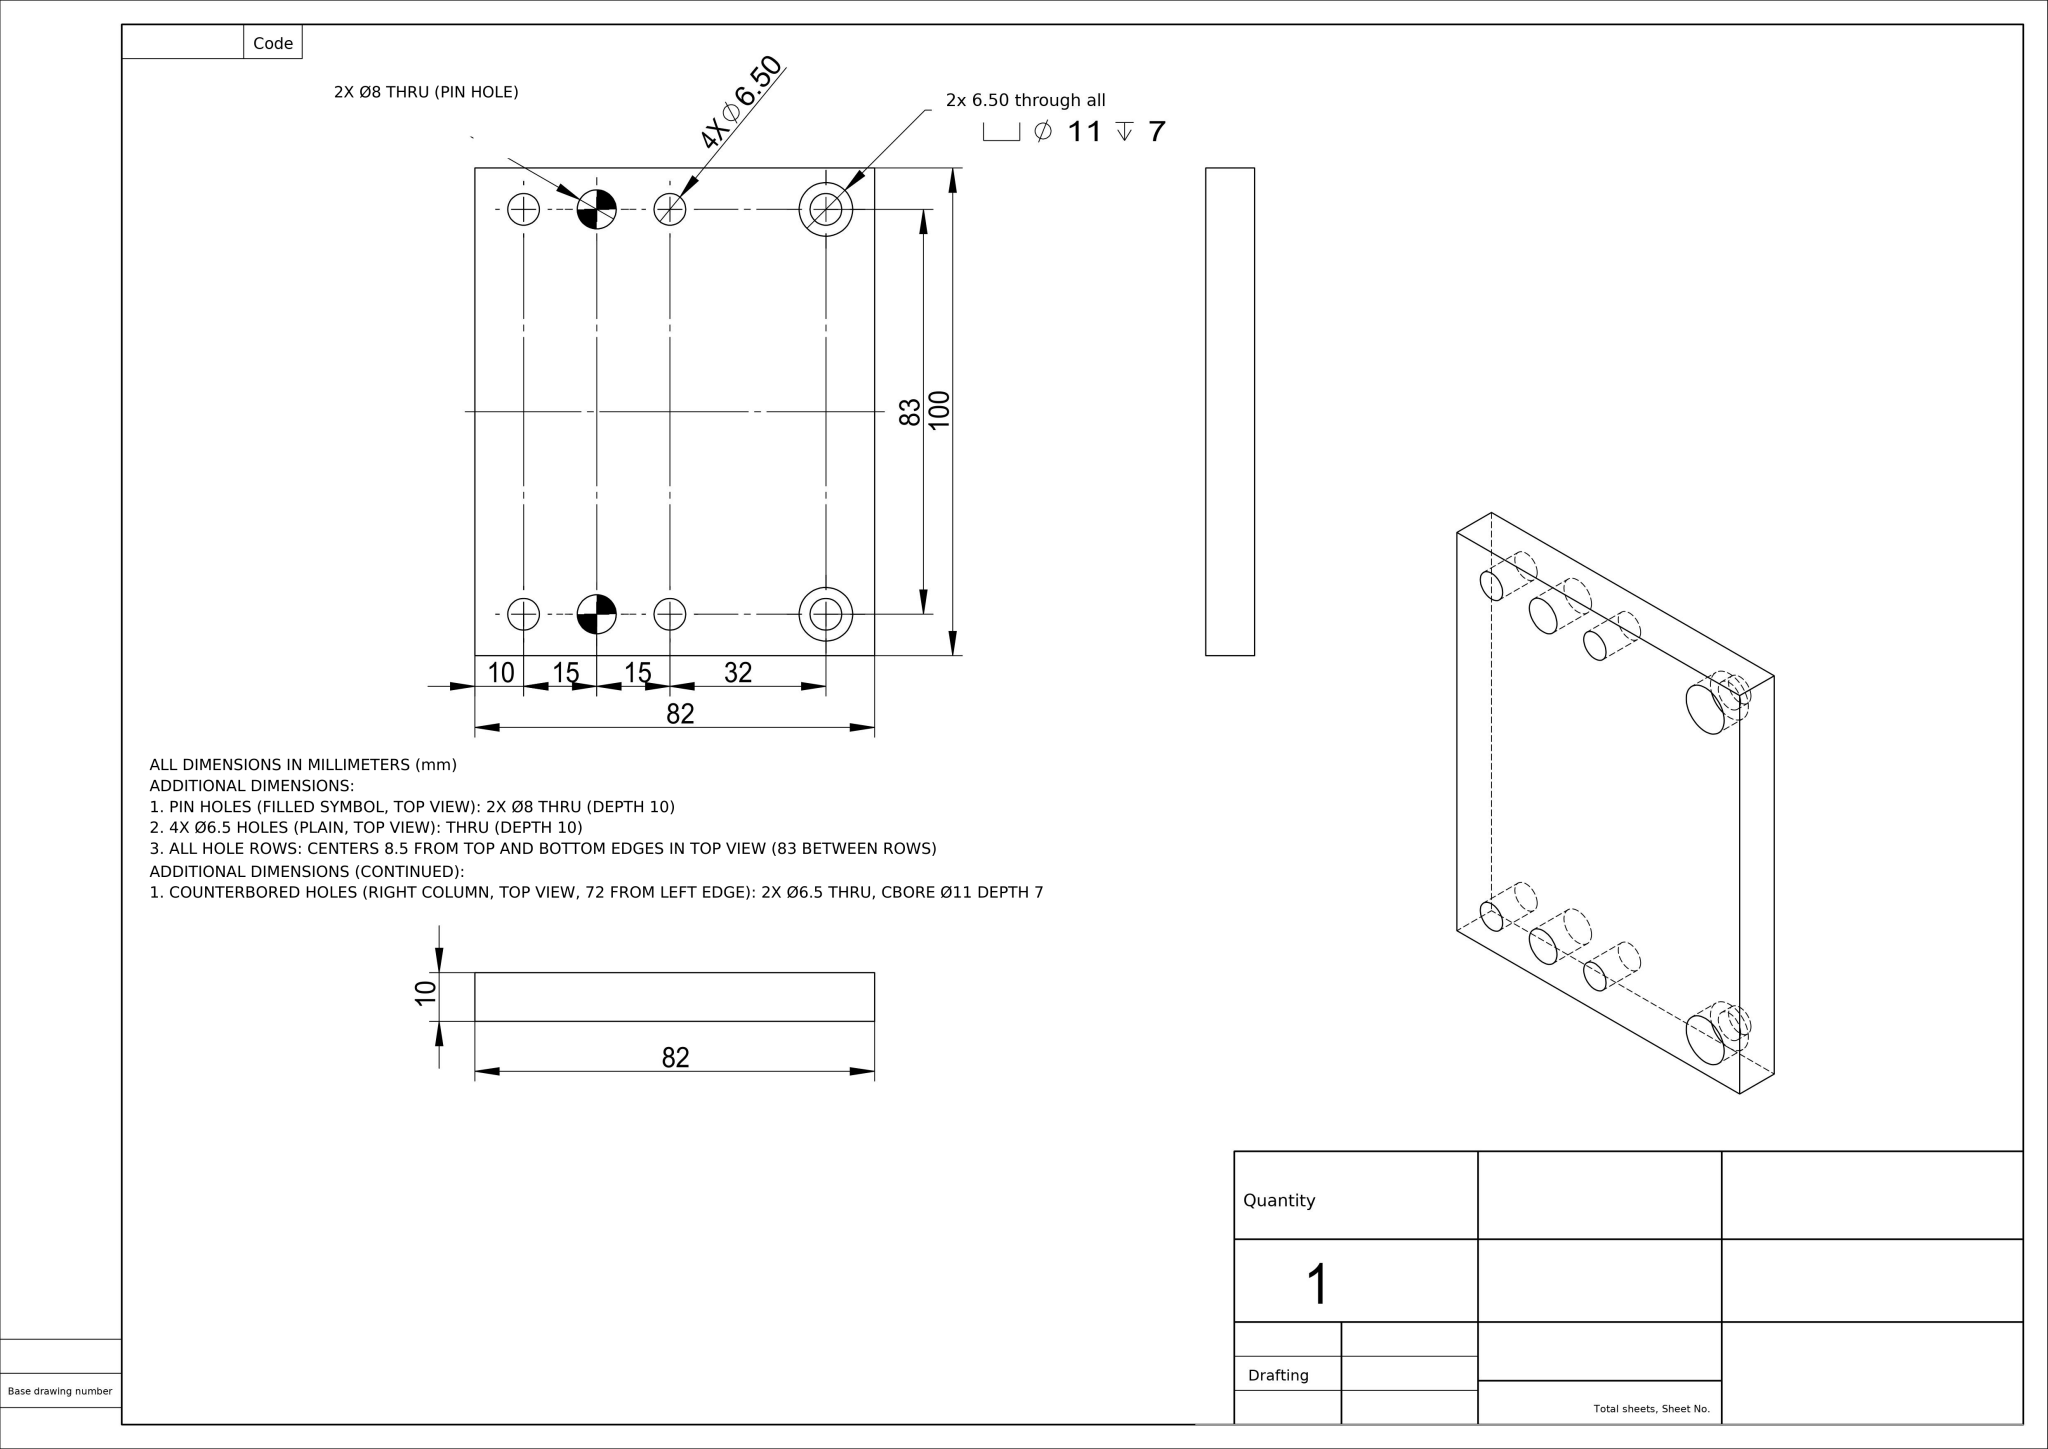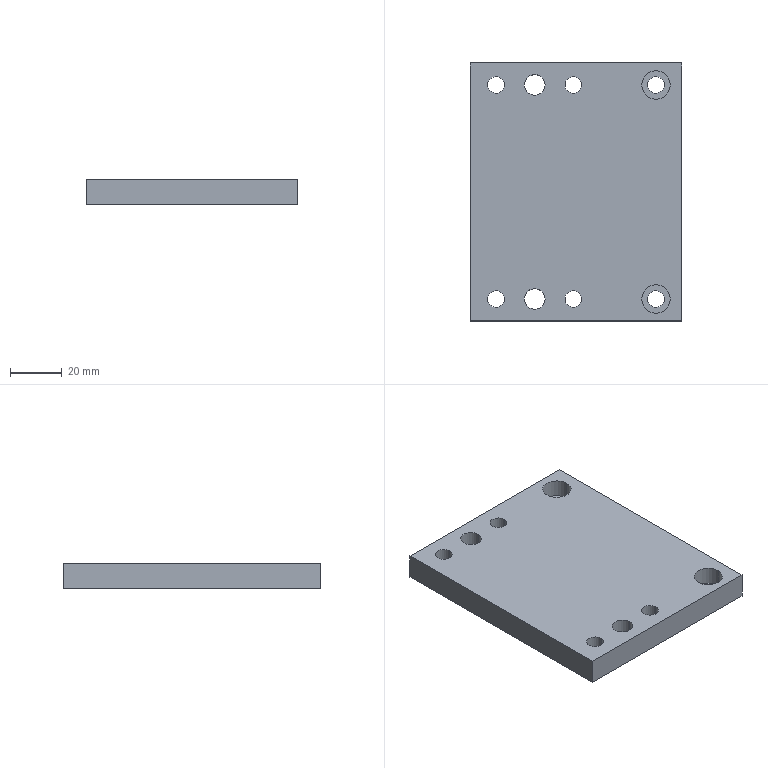Part | NX | mm | 1 solid | 28 faces | box 82 x 100 x 10 mm | volume 78138 mm3 | cylinder 20 | plane 8 | commonest cylinder face diameters 6.5 x12 11 x4 8 x4
STEP:
#1=COLOUR_RGB('',0.502,1.,1.);
#2=FILL_AREA_STYLE_COLOUR('',#1);
#3=FILL_AREA_STYLE('',(#2));
#4=SURFACE_STYLE_FILL_AREA(#3);
#5=SURFACE_SIDE_STYLE('',(#4));
#6=SURFACE_STYLE_USAGE(.BOTH.,#5);
#7=PRESENTATION_STYLE_ASSIGNMENT((#6));
#8=CARTESIAN_POINT('',(25.5,-41.5,-7.));
#9=VERTEX_POINT('',#8);
#10=CARTESIAN_POINT('',(36.5,-41.5,-7.));
#11=VERTEX_POINT('',#10);
#12=CARTESIAN_POINT('',(31.,-41.5,-7.));
#13=DIRECTION('',(0.,0.,1.));
#14=DIRECTION('',(1.,0.,0.));
#15=AXIS2_PLACEMENT_3D('',#12,#13,#14);
#16=CIRCLE('',#15,5.5);
#17=EDGE_CURVE('',#9,#11,#16,.T.);
#18=ORIENTED_EDGE('',*,*,#17,.F.);
#19=CARTESIAN_POINT('',(25.5,-41.5,-0.));
#20=VERTEX_POINT('',#19);
#21=CARTESIAN_POINT('',(25.5,-41.5,0.));
#22=DIRECTION('',(0.,0.,1.));
#23=VECTOR('',#22,1000.);
#24=LINE('',#21,#23);
#25=EDGE_CURVE('',#9,#20,#24,.T.);
#26=ORIENTED_EDGE('',*,*,#25,.T.);
#27=CARTESIAN_POINT('',(36.5,-41.5,-0.));
#28=VERTEX_POINT('',#27);
#29=CARTESIAN_POINT('',(31.,-41.5,-0.));
#30=DIRECTION('',(0.,0.,1.));
#31=DIRECTION('',(1.,0.,0.));
#32=AXIS2_PLACEMENT_3D('',#29,#30,#31);
#33=CIRCLE('',#32,5.5);
#34=EDGE_CURVE('',#20,#28,#33,.T.);
#35=ORIENTED_EDGE('',*,*,#34,.T.);
#36=CARTESIAN_POINT('',(36.5,-41.5,0.));
#37=DIRECTION('',(0.,0.,1.));
#38=VECTOR('',#37,1000.);
#39=LINE('',#36,#38);
#40=EDGE_CURVE('',#11,#28,#39,.T.);
#41=ORIENTED_EDGE('',*,*,#40,.F.);
#42=EDGE_LOOP('',(#18,#26,#35,#41));
#43=FACE_OUTER_BOUND('',#42,.T.);
#44=CARTESIAN_POINT('',(31.,-41.5,0.));
#45=DIRECTION('',(0.,0.,1.));
#46=DIRECTION('',(1.,0.,0.));
#47=AXIS2_PLACEMENT_3D('',#44,#45,#46);
#48=CYLINDRICAL_SURFACE('',#47,5.5);
#49=ADVANCED_FACE('',(#43),#48,.F.);
#50=CARTESIAN_POINT('',(27.75,-41.5,-10.));
#51=VERTEX_POINT('',#50);
#52=CARTESIAN_POINT('',(34.25,-41.5,-10.));
#53=VERTEX_POINT('',#52);
#54=CARTESIAN_POINT('',(31.,-41.5,-10.));
#55=DIRECTION('',(0.,0.,1.));
#56=DIRECTION('',(1.,0.,0.));
#57=AXIS2_PLACEMENT_3D('',#54,#55,#56);
#58=CIRCLE('',#57,3.25);
#59=EDGE_CURVE('',#51,#53,#58,.T.);
#60=ORIENTED_EDGE('',*,*,#59,.F.);
#61=CARTESIAN_POINT('',(27.75,-41.5,-7.));
#62=VERTEX_POINT('',#61);
#63=CARTESIAN_POINT('',(27.75,-41.5,0.));
#64=DIRECTION('',(0.,0.,1.));
#65=VECTOR('',#64,1000.);
#66=LINE('',#63,#65);
#67=EDGE_CURVE('',#51,#62,#66,.T.);
#68=ORIENTED_EDGE('',*,*,#67,.T.);
#69=CARTESIAN_POINT('',(34.25,-41.5,-7.));
#70=VERTEX_POINT('',#69);
#71=CARTESIAN_POINT('',(31.,-41.5,-7.));
#72=DIRECTION('',(0.,0.,1.));
#73=DIRECTION('',(1.,0.,0.));
#74=AXIS2_PLACEMENT_3D('',#71,#72,#73);
#75=CIRCLE('',#74,3.25);
#76=EDGE_CURVE('',#62,#70,#75,.T.);
#77=ORIENTED_EDGE('',*,*,#76,.T.);
#78=CARTESIAN_POINT('',(34.25,-41.5,0.));
#79=DIRECTION('',(0.,0.,1.));
#80=VECTOR('',#79,1000.);
#81=LINE('',#78,#80);
#82=EDGE_CURVE('',#53,#70,#81,.T.);
#83=ORIENTED_EDGE('',*,*,#82,.F.);
#84=EDGE_LOOP('',(#60,#68,#77,#83));
#85=FACE_OUTER_BOUND('',#84,.T.);
#86=CARTESIAN_POINT('',(31.,-41.5,0.));
#87=DIRECTION('',(0.,0.,1.));
#88=DIRECTION('',(1.,0.,0.));
#89=AXIS2_PLACEMENT_3D('',#86,#87,#88);
#90=CYLINDRICAL_SURFACE('',#89,3.25);
#91=ADVANCED_FACE('',(#85),#90,.F.);
#92=CARTESIAN_POINT('',(25.5,41.5,-7.));
#93=VERTEX_POINT('',#92);
#94=CARTESIAN_POINT('',(36.5,41.5,-7.));
#95=VERTEX_POINT('',#94);
#96=CARTESIAN_POINT('',(31.,41.5,-7.));
#97=DIRECTION('',(0.,0.,1.));
#98=DIRECTION('',(1.,0.,0.));
#99=AXIS2_PLACEMENT_3D('',#96,#97,#98);
#100=CIRCLE('',#99,5.5);
#101=EDGE_CURVE('',#93,#95,#100,.T.);
#102=ORIENTED_EDGE('',*,*,#101,.F.);
#103=CARTESIAN_POINT('',(25.5,41.5,-0.));
#104=VERTEX_POINT('',#103);
#105=CARTESIAN_POINT('',(25.5,41.5,0.));
#106=DIRECTION('',(0.,0.,1.));
#107=VECTOR('',#106,1000.);
#108=LINE('',#105,#107);
#109=EDGE_CURVE('',#93,#104,#108,.T.);
#110=ORIENTED_EDGE('',*,*,#109,.T.);
#111=CARTESIAN_POINT('',(36.5,41.5,-0.));
#112=VERTEX_POINT('',#111);
#113=CARTESIAN_POINT('',(31.,41.5,-0.));
#114=DIRECTION('',(0.,0.,1.));
#115=DIRECTION('',(1.,0.,0.));
#116=AXIS2_PLACEMENT_3D('',#113,#114,#115);
#117=CIRCLE('',#116,5.5);
#118=EDGE_CURVE('',#104,#112,#117,.T.);
#119=ORIENTED_EDGE('',*,*,#118,.T.);
#120=CARTESIAN_POINT('',(36.5,41.5,0.));
#121=DIRECTION('',(0.,0.,1.));
#122=VECTOR('',#121,1000.);
#123=LINE('',#120,#122);
#124=EDGE_CURVE('',#95,#112,#123,.T.);
#125=ORIENTED_EDGE('',*,*,#124,.F.);
#126=EDGE_LOOP('',(#102,#110,#119,#125));
#127=FACE_OUTER_BOUND('',#126,.T.);
#128=CARTESIAN_POINT('',(31.,41.5,0.));
#129=DIRECTION('',(0.,0.,1.));
#130=DIRECTION('',(1.,0.,0.));
#131=AXIS2_PLACEMENT_3D('',#128,#129,#130);
#132=CYLINDRICAL_SURFACE('',#131,5.5);
#133=ADVANCED_FACE('',(#127),#132,.F.);
#134=CARTESIAN_POINT('',(27.75,41.5,-10.));
#135=VERTEX_POINT('',#134);
#136=CARTESIAN_POINT('',(34.25,41.5,-10.));
#137=VERTEX_POINT('',#136);
#138=CARTESIAN_POINT('',(31.,41.5,-10.));
#139=DIRECTION('',(0.,0.,1.));
#140=DIRECTION('',(1.,0.,0.));
#141=AXIS2_PLACEMENT_3D('',#138,#139,#140);
#142=CIRCLE('',#141,3.25);
#143=EDGE_CURVE('',#135,#137,#142,.T.);
#144=ORIENTED_EDGE('',*,*,#143,.F.);
#145=CARTESIAN_POINT('',(27.75,41.5,-7.));
#146=VERTEX_POINT('',#145);
#147=CARTESIAN_POINT('',(27.75,41.5,0.));
#148=DIRECTION('',(0.,0.,1.));
#149=VECTOR('',#148,1000.);
#150=LINE('',#147,#149);
#151=EDGE_CURVE('',#135,#146,#150,.T.);
#152=ORIENTED_EDGE('',*,*,#151,.T.);
#153=CARTESIAN_POINT('',(34.25,41.5,-7.));
#154=VERTEX_POINT('',#153);
#155=CARTESIAN_POINT('',(31.,41.5,-7.));
#156=DIRECTION('',(0.,0.,1.));
#157=DIRECTION('',(1.,0.,0.));
#158=AXIS2_PLACEMENT_3D('',#155,#156,#157);
#159=CIRCLE('',#158,3.25);
#160=EDGE_CURVE('',#146,#154,#159,.T.);
#161=ORIENTED_EDGE('',*,*,#160,.T.);
#162=CARTESIAN_POINT('',(34.25,41.5,0.));
#163=DIRECTION('',(0.,0.,1.));
#164=VECTOR('',#163,1000.);
#165=LINE('',#162,#164);
#166=EDGE_CURVE('',#137,#154,#165,.T.);
#167=ORIENTED_EDGE('',*,*,#166,.F.);
#168=EDGE_LOOP('',(#144,#152,#161,#167));
#169=FACE_OUTER_BOUND('',#168,.T.);
#170=CARTESIAN_POINT('',(31.,41.5,0.));
#171=DIRECTION('',(0.,0.,1.));
#172=DIRECTION('',(1.,0.,0.));
#173=AXIS2_PLACEMENT_3D('',#170,#171,#172);
#174=CYLINDRICAL_SURFACE('',#173,3.25);
#175=ADVANCED_FACE('',(#169),#174,.F.);
#176=CARTESIAN_POINT('',(-20.,-41.5,-10.));
#177=VERTEX_POINT('',#176);
#178=CARTESIAN_POINT('',(-12.,-41.5,-10.));
#179=VERTEX_POINT('',#178);
#180=CARTESIAN_POINT('',(-16.,-41.5,-10.));
#181=DIRECTION('',(0.,0.,1.));
#182=DIRECTION('',(1.,0.,0.));
#183=AXIS2_PLACEMENT_3D('',#180,#181,#182);
#184=CIRCLE('',#183,4.);
#185=EDGE_CURVE('',#177,#179,#184,.T.);
#186=ORIENTED_EDGE('',*,*,#185,.F.);
#187=CARTESIAN_POINT('',(-20.,-41.5,0.));
#188=VERTEX_POINT('',#187);
#189=CARTESIAN_POINT('',(-20.,-41.5,0.));
#190=DIRECTION('',(0.,0.,1.));
#191=VECTOR('',#190,1000.);
#192=LINE('',#189,#191);
#193=EDGE_CURVE('',#177,#188,#192,.T.);
#194=ORIENTED_EDGE('',*,*,#193,.T.);
#195=CARTESIAN_POINT('',(-12.,-41.5,0.));
#196=VERTEX_POINT('',#195);
#197=CARTESIAN_POINT('',(-16.,-41.5,0.));
#198=DIRECTION('',(0.,0.,1.));
#199=DIRECTION('',(1.,0.,0.));
#200=AXIS2_PLACEMENT_3D('',#197,#198,#199);
#201=CIRCLE('',#200,4.);
#202=EDGE_CURVE('',#188,#196,#201,.T.);
#203=ORIENTED_EDGE('',*,*,#202,.T.);
#204=CARTESIAN_POINT('',(-12.,-41.5,0.));
#205=DIRECTION('',(0.,0.,1.));
#206=VECTOR('',#205,1000.);
#207=LINE('',#204,#206);
#208=EDGE_CURVE('',#179,#196,#207,.T.);
#209=ORIENTED_EDGE('',*,*,#208,.F.);
#210=EDGE_LOOP('',(#186,#194,#203,#209));
#211=FACE_OUTER_BOUND('',#210,.T.);
#212=CARTESIAN_POINT('',(-16.,-41.5,0.));
#213=DIRECTION('',(0.,0.,1.));
#214=DIRECTION('',(1.,0.,0.));
#215=AXIS2_PLACEMENT_3D('',#212,#213,#214);
#216=CYLINDRICAL_SURFACE('',#215,4.);
#217=ADVANCED_FACE('',(#211),#216,.F.);
#218=CARTESIAN_POINT('',(-20.,41.5,-10.));
#219=VERTEX_POINT('',#218);
#220=CARTESIAN_POINT('',(-12.,41.5,-10.));
#221=VERTEX_POINT('',#220);
#222=CARTESIAN_POINT('',(-16.,41.5,-10.));
#223=DIRECTION('',(0.,0.,1.));
#224=DIRECTION('',(1.,0.,0.));
#225=AXIS2_PLACEMENT_3D('',#222,#223,#224);
#226=CIRCLE('',#225,4.);
#227=EDGE_CURVE('',#219,#221,#226,.T.);
#228=ORIENTED_EDGE('',*,*,#227,.F.);
#229=CARTESIAN_POINT('',(-20.,41.5,0.));
#230=VERTEX_POINT('',#229);
#231=CARTESIAN_POINT('',(-20.,41.5,0.));
#232=DIRECTION('',(0.,0.,1.));
#233=VECTOR('',#232,1000.);
#234=LINE('',#231,#233);
#235=EDGE_CURVE('',#219,#230,#234,.T.);
#236=ORIENTED_EDGE('',*,*,#235,.T.);
#237=CARTESIAN_POINT('',(-12.,41.5,0.));
#238=VERTEX_POINT('',#237);
#239=CARTESIAN_POINT('',(-16.,41.5,0.));
#240=DIRECTION('',(0.,0.,1.));
#241=DIRECTION('',(1.,0.,0.));
#242=AXIS2_PLACEMENT_3D('',#239,#240,#241);
#243=CIRCLE('',#242,4.);
#244=EDGE_CURVE('',#230,#238,#243,.T.);
#245=ORIENTED_EDGE('',*,*,#244,.T.);
#246=CARTESIAN_POINT('',(-12.,41.5,0.));
#247=DIRECTION('',(0.,0.,1.));
#248=VECTOR('',#247,1000.);
#249=LINE('',#246,#248);
#250=EDGE_CURVE('',#221,#238,#249,.T.);
#251=ORIENTED_EDGE('',*,*,#250,.F.);
#252=EDGE_LOOP('',(#228,#236,#245,#251));
#253=FACE_OUTER_BOUND('',#252,.T.);
#254=CARTESIAN_POINT('',(-16.,41.5,0.));
#255=DIRECTION('',(0.,0.,1.));
#256=DIRECTION('',(1.,0.,0.));
#257=AXIS2_PLACEMENT_3D('',#254,#255,#256);
#258=CYLINDRICAL_SURFACE('',#257,4.);
#259=ADVANCED_FACE('',(#253),#258,.F.);
#260=CARTESIAN_POINT('',(-4.25,41.5,-10.));
#261=VERTEX_POINT('',#260);
#262=CARTESIAN_POINT('',(2.25,41.5,-10.));
#263=VERTEX_POINT('',#262);
#264=CARTESIAN_POINT('',(-1.,41.5,-10.));
#265=DIRECTION('',(0.,0.,1.));
#266=DIRECTION('',(1.,0.,0.));
#267=AXIS2_PLACEMENT_3D('',#264,#265,#266);
#268=CIRCLE('',#267,3.25);
#269=EDGE_CURVE('',#261,#263,#268,.T.);
#270=ORIENTED_EDGE('',*,*,#269,.F.);
#271=CARTESIAN_POINT('',(-4.25,41.5,0.));
#272=VERTEX_POINT('',#271);
#273=CARTESIAN_POINT('',(-4.25,41.5,-10.));
#274=DIRECTION('',(0.,0.,1.));
#275=VECTOR('',#274,1000.);
#276=LINE('',#273,#275);
#277=EDGE_CURVE('',#261,#272,#276,.T.);
#278=ORIENTED_EDGE('',*,*,#277,.T.);
#279=CARTESIAN_POINT('',(2.25,41.5,0.));
#280=VERTEX_POINT('',#279);
#281=CARTESIAN_POINT('',(-1.,41.5,0.));
#282=DIRECTION('',(0.,0.,1.));
#283=DIRECTION('',(1.,0.,0.));
#284=AXIS2_PLACEMENT_3D('',#281,#282,#283);
#285=CIRCLE('',#284,3.25);
#286=EDGE_CURVE('',#272,#280,#285,.T.);
#287=ORIENTED_EDGE('',*,*,#286,.T.);
#288=CARTESIAN_POINT('',(2.25,41.5,-10.));
#289=DIRECTION('',(0.,0.,1.));
#290=VECTOR('',#289,1000.);
#291=LINE('',#288,#290);
#292=EDGE_CURVE('',#263,#280,#291,.T.);
#293=ORIENTED_EDGE('',*,*,#292,.F.);
#294=EDGE_LOOP('',(#270,#278,#287,#293));
#295=FACE_OUTER_BOUND('',#294,.T.);
#296=CARTESIAN_POINT('',(-1.,41.5,-10.));
#297=DIRECTION('',(0.,0.,1.));
#298=DIRECTION('',(1.,0.,0.));
#299=AXIS2_PLACEMENT_3D('',#296,#297,#298);
#300=CYLINDRICAL_SURFACE('',#299,3.25);
#301=ADVANCED_FACE('',(#295),#300,.F.);
#302=CARTESIAN_POINT('',(-34.25,41.5,-10.));
#303=VERTEX_POINT('',#302);
#304=CARTESIAN_POINT('',(-27.75,41.5,-10.));
#305=VERTEX_POINT('',#304);
#306=CARTESIAN_POINT('',(-31.,41.5,-10.));
#307=DIRECTION('',(0.,0.,1.));
#308=DIRECTION('',(1.,0.,0.));
#309=AXIS2_PLACEMENT_3D('',#306,#307,#308);
#310=CIRCLE('',#309,3.25);
#311=EDGE_CURVE('',#303,#305,#310,.T.);
#312=ORIENTED_EDGE('',*,*,#311,.F.);
#313=CARTESIAN_POINT('',(-34.25,41.5,0.));
#314=VERTEX_POINT('',#313);
#315=CARTESIAN_POINT('',(-34.25,41.5,-10.));
#316=DIRECTION('',(0.,0.,1.));
#317=VECTOR('',#316,1000.);
#318=LINE('',#315,#317);
#319=EDGE_CURVE('',#303,#314,#318,.T.);
#320=ORIENTED_EDGE('',*,*,#319,.T.);
#321=CARTESIAN_POINT('',(-27.75,41.5,0.));
#322=VERTEX_POINT('',#321);
#323=CARTESIAN_POINT('',(-31.,41.5,0.));
#324=DIRECTION('',(0.,0.,1.));
#325=DIRECTION('',(1.,0.,0.));
#326=AXIS2_PLACEMENT_3D('',#323,#324,#325);
#327=CIRCLE('',#326,3.25);
#328=EDGE_CURVE('',#314,#322,#327,.T.);
#329=ORIENTED_EDGE('',*,*,#328,.T.);
#330=CARTESIAN_POINT('',(-27.75,41.5,-10.));
#331=DIRECTION('',(0.,0.,1.));
#332=VECTOR('',#331,1000.);
#333=LINE('',#330,#332);
#334=EDGE_CURVE('',#305,#322,#333,.T.);
#335=ORIENTED_EDGE('',*,*,#334,.F.);
#336=EDGE_LOOP('',(#312,#320,#329,#335));
#337=FACE_OUTER_BOUND('',#336,.T.);
#338=CARTESIAN_POINT('',(-31.,41.5,-10.));
#339=DIRECTION('',(0.,0.,1.));
#340=DIRECTION('',(1.,0.,0.));
#341=AXIS2_PLACEMENT_3D('',#338,#339,#340);
#342=CYLINDRICAL_SURFACE('',#341,3.25);
#343=ADVANCED_FACE('',(#337),#342,.F.);
#344=CARTESIAN_POINT('',(-4.25,-41.5,-10.));
#345=VERTEX_POINT('',#344);
#346=CARTESIAN_POINT('',(2.25,-41.5,-10.));
#347=VERTEX_POINT('',#346);
#348=CARTESIAN_POINT('',(-1.,-41.5,-10.));
#349=DIRECTION('',(0.,0.,1.));
#350=DIRECTION('',(1.,0.,0.));
#351=AXIS2_PLACEMENT_3D('',#348,#349,#350);
#352=CIRCLE('',#351,3.25);
#353=EDGE_CURVE('',#345,#347,#352,.T.);
#354=ORIENTED_EDGE('',*,*,#353,.F.);
#355=CARTESIAN_POINT('',(-4.25,-41.5,0.));
#356=VERTEX_POINT('',#355);
#357=CARTESIAN_POINT('',(-4.25,-41.5,-10.));
#358=DIRECTION('',(0.,0.,1.));
#359=VECTOR('',#358,1000.);
#360=LINE('',#357,#359);
#361=EDGE_CURVE('',#345,#356,#360,.T.);
#362=ORIENTED_EDGE('',*,*,#361,.T.);
#363=CARTESIAN_POINT('',(2.25,-41.5,0.));
#364=VERTEX_POINT('',#363);
#365=CARTESIAN_POINT('',(-1.,-41.5,0.));
#366=DIRECTION('',(0.,0.,1.));
#367=DIRECTION('',(1.,0.,0.));
#368=AXIS2_PLACEMENT_3D('',#365,#366,#367);
#369=CIRCLE('',#368,3.25);
#370=EDGE_CURVE('',#356,#364,#369,.T.);
#371=ORIENTED_EDGE('',*,*,#370,.T.);
#372=CARTESIAN_POINT('',(2.25,-41.5,-10.));
#373=DIRECTION('',(0.,0.,1.));
#374=VECTOR('',#373,1000.);
#375=LINE('',#372,#374);
#376=EDGE_CURVE('',#347,#364,#375,.T.);
#377=ORIENTED_EDGE('',*,*,#376,.F.);
#378=EDGE_LOOP('',(#354,#362,#371,#377));
#379=FACE_OUTER_BOUND('',#378,.T.);
#380=CARTESIAN_POINT('',(-1.,-41.5,-10.));
#381=DIRECTION('',(0.,0.,1.));
#382=DIRECTION('',(1.,0.,0.));
#383=AXIS2_PLACEMENT_3D('',#380,#381,#382);
#384=CYLINDRICAL_SURFACE('',#383,3.25);
#385=ADVANCED_FACE('',(#379),#384,.F.);
#386=CARTESIAN_POINT('',(-34.25,-41.5,-10.));
#387=VERTEX_POINT('',#386);
#388=CARTESIAN_POINT('',(-27.75,-41.5,-10.));
#389=VERTEX_POINT('',#388);
#390=CARTESIAN_POINT('',(-31.,-41.5,-10.));
#391=DIRECTION('',(0.,0.,1.));
#392=DIRECTION('',(1.,0.,0.));
#393=AXIS2_PLACEMENT_3D('',#390,#391,#392);
#394=CIRCLE('',#393,3.25);
#395=EDGE_CURVE('',#387,#389,#394,.T.);
#396=ORIENTED_EDGE('',*,*,#395,.F.);
#397=CARTESIAN_POINT('',(-34.25,-41.5,0.));
#398=VERTEX_POINT('',#397);
#399=CARTESIAN_POINT('',(-34.25,-41.5,-10.));
#400=DIRECTION('',(0.,0.,1.));
#401=VECTOR('',#400,1000.);
#402=LINE('',#399,#401);
#403=EDGE_CURVE('',#387,#398,#402,.T.);
#404=ORIENTED_EDGE('',*,*,#403,.T.);
#405=CARTESIAN_POINT('',(-27.75,-41.5,0.));
#406=VERTEX_POINT('',#405);
#407=CARTESIAN_POINT('',(-31.,-41.5,0.));
#408=DIRECTION('',(0.,0.,1.));
#409=DIRECTION('',(1.,0.,0.));
#410=AXIS2_PLACEMENT_3D('',#407,#408,#409);
#411=CIRCLE('',#410,3.25);
#412=EDGE_CURVE('',#398,#406,#411,.T.);
#413=ORIENTED_EDGE('',*,*,#412,.T.);
#414=CARTESIAN_POINT('',(-27.75,-41.5,-10.));
#415=DIRECTION('',(0.,0.,1.));
#416=VECTOR('',#415,1000.);
#417=LINE('',#414,#416);
#418=EDGE_CURVE('',#389,#406,#417,.T.);
#419=ORIENTED_EDGE('',*,*,#418,.F.);
#420=EDGE_LOOP('',(#396,#404,#413,#419));
#421=FACE_OUTER_BOUND('',#420,.T.);
#422=CARTESIAN_POINT('',(-31.,-41.5,-10.));
#423=DIRECTION('',(0.,0.,1.));
#424=DIRECTION('',(1.,0.,0.));
#425=AXIS2_PLACEMENT_3D('',#422,#423,#424);
#426=CYLINDRICAL_SURFACE('',#425,3.25);
#427=ADVANCED_FACE('',(#421),#426,.F.);
#428=CARTESIAN_POINT('',(-41.,50.,0.));
#429=VERTEX_POINT('',#428);
#430=CARTESIAN_POINT('',(-41.,-50.,0.));
#431=VERTEX_POINT('',#430);
#432=CARTESIAN_POINT('',(-41.,50.,0.));
#433=DIRECTION('',(0.,-1.,0.));
#434=VECTOR('',#433,1000.);
#435=LINE('',#432,#434);
#436=EDGE_CURVE('',#429,#431,#435,.T.);
#437=ORIENTED_EDGE('',*,*,#436,.F.);
#438=CARTESIAN_POINT('',(-41.,50.,-10.));
#439=VERTEX_POINT('',#438);
#440=CARTESIAN_POINT('',(-41.,50.,-10.));
#441=DIRECTION('',(0.,0.,1.));
#442=VECTOR('',#441,1000.);
#443=LINE('',#440,#442);
#444=EDGE_CURVE('',#439,#429,#443,.T.);
#445=ORIENTED_EDGE('',*,*,#444,.F.);
#446=CARTESIAN_POINT('',(-41.,-50.,-10.));
#447=VERTEX_POINT('',#446);
#448=CARTESIAN_POINT('',(-41.,50.,-10.));
#449=DIRECTION('',(0.,-1.,0.));
#450=VECTOR('',#449,1000.);
#451=LINE('',#448,#450);
#452=EDGE_CURVE('',#439,#447,#451,.T.);
#453=ORIENTED_EDGE('',*,*,#452,.T.);
#454=CARTESIAN_POINT('',(-41.,-50.,-10.));
#455=DIRECTION('',(0.,0.,1.));
#456=VECTOR('',#455,1000.);
#457=LINE('',#454,#456);
#458=EDGE_CURVE('',#447,#431,#457,.T.);
#459=ORIENTED_EDGE('',*,*,#458,.T.);
#460=EDGE_LOOP('',(#437,#445,#453,#459));
#461=FACE_OUTER_BOUND('',#460,.T.);
#462=CARTESIAN_POINT('',(-41.,50.,-10.));
#463=DIRECTION('',(-1.,0.,0.));
#464=DIRECTION('',(0.,0.,1.));
#465=AXIS2_PLACEMENT_3D('',#462,#463,#464);
#466=PLANE('',#465);
#467=ADVANCED_FACE('',(#461),#466,.T.);
#468=CARTESIAN_POINT('',(41.,50.,0.));
#469=VERTEX_POINT('',#468);
#470=CARTESIAN_POINT('',(-41.,50.,0.));
#471=DIRECTION('',(-1.,0.,0.));
#472=VECTOR('',#471,1000.);
#473=LINE('',#470,#472);
#474=EDGE_CURVE('',#469,#429,#473,.T.);
#475=ORIENTED_EDGE('',*,*,#474,.F.);
#476=CARTESIAN_POINT('',(41.,50.,-10.));
#477=VERTEX_POINT('',#476);
#478=CARTESIAN_POINT('',(41.,50.,-10.));
#479=DIRECTION('',(0.,0.,1.));
#480=VECTOR('',#479,1000.);
#481=LINE('',#478,#480);
#482=EDGE_CURVE('',#477,#469,#481,.T.);
#483=ORIENTED_EDGE('',*,*,#482,.F.);
#484=CARTESIAN_POINT('',(-41.,50.,-10.));
#485=DIRECTION('',(-1.,0.,0.));
#486=VECTOR('',#485,1000.);
#487=LINE('',#484,#486);
#488=EDGE_CURVE('',#477,#439,#487,.T.);
#489=ORIENTED_EDGE('',*,*,#488,.T.);
#490=ORIENTED_EDGE('',*,*,#444,.T.);
#491=EDGE_LOOP('',(#475,#483,#489,#490));
#492=FACE_OUTER_BOUND('',#491,.T.);
#493=CARTESIAN_POINT('',(-41.,50.,-10.));
#494=DIRECTION('',(0.,1.,0.));
#495=DIRECTION('',(0.,0.,1.));
#496=AXIS2_PLACEMENT_3D('',#493,#494,#495);
#497=PLANE('',#496);
#498=ADVANCED_FACE('',(#492),#497,.T.);
#499=CARTESIAN_POINT('',(41.,-50.,0.));
#500=VERTEX_POINT('',#499);
#501=CARTESIAN_POINT('',(41.,50.,0.));
#502=DIRECTION('',(0.,1.,0.));
#503=VECTOR('',#502,1000.);
#504=LINE('',#501,#503);
#505=EDGE_CURVE('',#500,#469,#504,.T.);
#506=ORIENTED_EDGE('',*,*,#505,.F.);
#507=CARTESIAN_POINT('',(41.,-50.,-10.));
#508=VERTEX_POINT('',#507);
#509=CARTESIAN_POINT('',(41.,-50.,-10.));
#510=DIRECTION('',(0.,0.,1.));
#511=VECTOR('',#510,1000.);
#512=LINE('',#509,#511);
#513=EDGE_CURVE('',#508,#500,#512,.T.);
#514=ORIENTED_EDGE('',*,*,#513,.F.);
#515=CARTESIAN_POINT('',(41.,50.,-10.));
#516=DIRECTION('',(0.,1.,0.));
#517=VECTOR('',#516,1000.);
#518=LINE('',#515,#517);
#519=EDGE_CURVE('',#508,#477,#518,.T.);
#520=ORIENTED_EDGE('',*,*,#519,.T.);
#521=ORIENTED_EDGE('',*,*,#482,.T.);
#522=EDGE_LOOP('',(#506,#514,#520,#521));
#523=FACE_OUTER_BOUND('',#522,.T.);
#524=CARTESIAN_POINT('',(41.,50.,-10.));
#525=DIRECTION('',(1.,0.,0.));
#526=DIRECTION('',(0.,0.,-1.));
#527=AXIS2_PLACEMENT_3D('',#524,#525,#526);
#528=PLANE('',#527);
#529=ADVANCED_FACE('',(#523),#528,.T.);
#530=CARTESIAN_POINT('',(-41.,-50.,0.));
#531=DIRECTION('',(1.,0.,0.));
#532=VECTOR('',#531,1000.);
#533=LINE('',#530,#532);
#534=EDGE_CURVE('',#431,#500,#533,.T.);
#535=ORIENTED_EDGE('',*,*,#534,.F.);
#536=ORIENTED_EDGE('',*,*,#458,.F.);
#537=CARTESIAN_POINT('',(-41.,-50.,-10.));
#538=DIRECTION('',(1.,0.,0.));
#539=VECTOR('',#538,1000.);
#540=LINE('',#537,#539);
#541=EDGE_CURVE('',#447,#508,#540,.T.);
#542=ORIENTED_EDGE('',*,*,#541,.T.);
#543=ORIENTED_EDGE('',*,*,#513,.T.);
#544=EDGE_LOOP('',(#535,#536,#542,#543));
#545=FACE_OUTER_BOUND('',#544,.T.);
#546=CARTESIAN_POINT('',(-41.,-50.,-10.));
#547=DIRECTION('',(0.,-1.,0.));
#548=DIRECTION('',(0.,0.,-1.));
#549=AXIS2_PLACEMENT_3D('',#546,#547,#548);
#550=PLANE('',#549);
#551=ADVANCED_FACE('',(#545),#550,.T.);
#552=CARTESIAN_POINT('',(31.,-41.5,-10.));
#553=DIRECTION('',(0.,0.,1.));
#554=DIRECTION('',(1.,0.,0.));
#555=AXIS2_PLACEMENT_3D('',#552,#553,#554);
#556=CIRCLE('',#555,3.25);
#557=EDGE_CURVE('',#53,#51,#556,.T.);
#558=ORIENTED_EDGE('',*,*,#557,.T.);
#559=ORIENTED_EDGE('',*,*,#59,.T.);
#560=EDGE_LOOP('',(#558,#559));
#561=FACE_BOUND('',#560,.T.);
#562=CARTESIAN_POINT('',(31.,41.5,-10.));
#563=DIRECTION('',(0.,0.,1.));
#564=DIRECTION('',(1.,0.,0.));
#565=AXIS2_PLACEMENT_3D('',#562,#563,#564);
#566=CIRCLE('',#565,3.25);
#567=EDGE_CURVE('',#137,#135,#566,.T.);
#568=ORIENTED_EDGE('',*,*,#567,.T.);
#569=ORIENTED_EDGE('',*,*,#143,.T.);
#570=EDGE_LOOP('',(#568,#569));
#571=FACE_BOUND('',#570,.T.);
#572=CARTESIAN_POINT('',(-16.,-41.5,-10.));
#573=DIRECTION('',(0.,0.,1.));
#574=DIRECTION('',(1.,0.,0.));
#575=AXIS2_PLACEMENT_3D('',#572,#573,#574);
#576=CIRCLE('',#575,4.);
#577=EDGE_CURVE('',#179,#177,#576,.T.);
#578=ORIENTED_EDGE('',*,*,#577,.T.);
#579=ORIENTED_EDGE('',*,*,#185,.T.);
#580=EDGE_LOOP('',(#578,#579));
#581=FACE_BOUND('',#580,.T.);
#582=CARTESIAN_POINT('',(-16.,41.5,-10.));
#583=DIRECTION('',(0.,0.,1.));
#584=DIRECTION('',(1.,0.,0.));
#585=AXIS2_PLACEMENT_3D('',#582,#583,#584);
#586=CIRCLE('',#585,4.);
#587=EDGE_CURVE('',#221,#219,#586,.T.);
#588=ORIENTED_EDGE('',*,*,#587,.T.);
#589=ORIENTED_EDGE('',*,*,#227,.T.);
#590=EDGE_LOOP('',(#588,#589));
#591=FACE_BOUND('',#590,.T.);
#592=CARTESIAN_POINT('',(-1.,41.5,-10.));
#593=DIRECTION('',(0.,0.,1.));
#594=DIRECTION('',(1.,0.,0.));
#595=AXIS2_PLACEMENT_3D('',#592,#593,#594);
#596=CIRCLE('',#595,3.25);
#597=EDGE_CURVE('',#263,#261,#596,.T.);
#598=ORIENTED_EDGE('',*,*,#597,.T.);
#599=ORIENTED_EDGE('',*,*,#269,.T.);
#600=EDGE_LOOP('',(#598,#599));
#601=FACE_BOUND('',#600,.T.);
#602=CARTESIAN_POINT('',(-31.,41.5,-10.));
#603=DIRECTION('',(0.,0.,1.));
#604=DIRECTION('',(1.,0.,0.));
#605=AXIS2_PLACEMENT_3D('',#602,#603,#604);
#606=CIRCLE('',#605,3.25);
#607=EDGE_CURVE('',#305,#303,#606,.T.);
#608=ORIENTED_EDGE('',*,*,#607,.T.);
#609=ORIENTED_EDGE('',*,*,#311,.T.);
#610=EDGE_LOOP('',(#608,#609));
#611=FACE_BOUND('',#610,.T.);
#612=CARTESIAN_POINT('',(-1.,-41.5,-10.));
#613=DIRECTION('',(0.,0.,1.));
#614=DIRECTION('',(1.,0.,0.));
#615=AXIS2_PLACEMENT_3D('',#612,#613,#614);
#616=CIRCLE('',#615,3.25);
#617=EDGE_CURVE('',#347,#345,#616,.T.);
#618=ORIENTED_EDGE('',*,*,#617,.T.);
#619=ORIENTED_EDGE('',*,*,#353,.T.);
#620=EDGE_LOOP('',(#618,#619));
#621=FACE_BOUND('',#620,.T.);
#622=CARTESIAN_POINT('',(-31.,-41.5,-10.));
#623=DIRECTION('',(0.,0.,1.));
#624=DIRECTION('',(1.,0.,0.));
#625=AXIS2_PLACEMENT_3D('',#622,#623,#624);
#626=CIRCLE('',#625,3.25);
#627=EDGE_CURVE('',#389,#387,#626,.T.);
#628=ORIENTED_EDGE('',*,*,#627,.T.);
#629=ORIENTED_EDGE('',*,*,#395,.T.);
#630=EDGE_LOOP('',(#628,#629));
#631=FACE_BOUND('',#630,.T.);
#632=ORIENTED_EDGE('',*,*,#452,.F.);
#633=ORIENTED_EDGE('',*,*,#488,.F.);
#634=ORIENTED_EDGE('',*,*,#519,.F.);
#635=ORIENTED_EDGE('',*,*,#541,.F.);
#636=EDGE_LOOP('',(#632,#633,#634,#635));
#637=FACE_OUTER_BOUND('',#636,.T.);
#638=CARTESIAN_POINT('',(0.,0.,-10.));
#639=DIRECTION('',(0.,0.,1.));
#640=DIRECTION('',(1.,0.,0.));
#641=AXIS2_PLACEMENT_3D('',#638,#639,#640);
#642=PLANE('',#641);
#643=ADVANCED_FACE('',(#561,#571,#581,#591,#601,#611,#621,#631,#637),#642,.F.);
#644=CARTESIAN_POINT('',(31.,-41.5,-0.));
#645=DIRECTION('',(0.,0.,1.));
#646=DIRECTION('',(1.,0.,0.));
#647=AXIS2_PLACEMENT_3D('',#644,#645,#646);
#648=CIRCLE('',#647,5.5);
#649=EDGE_CURVE('',#28,#20,#648,.T.);
#650=ORIENTED_EDGE('',*,*,#649,.F.);
#651=ORIENTED_EDGE('',*,*,#34,.F.);
#652=EDGE_LOOP('',(#650,#651));
#653=FACE_BOUND('',#652,.T.);
#654=CARTESIAN_POINT('',(31.,41.5,-0.));
#655=DIRECTION('',(0.,0.,1.));
#656=DIRECTION('',(1.,0.,0.));
#657=AXIS2_PLACEMENT_3D('',#654,#655,#656);
#658=CIRCLE('',#657,5.5);
#659=EDGE_CURVE('',#112,#104,#658,.T.);
#660=ORIENTED_EDGE('',*,*,#659,.F.);
#661=ORIENTED_EDGE('',*,*,#118,.F.);
#662=EDGE_LOOP('',(#660,#661));
#663=FACE_BOUND('',#662,.T.);
#664=CARTESIAN_POINT('',(-16.,-41.5,0.));
#665=DIRECTION('',(0.,0.,1.));
#666=DIRECTION('',(1.,0.,0.));
#667=AXIS2_PLACEMENT_3D('',#664,#665,#666);
#668=CIRCLE('',#667,4.);
#669=EDGE_CURVE('',#196,#188,#668,.T.);
#670=ORIENTED_EDGE('',*,*,#669,.F.);
#671=ORIENTED_EDGE('',*,*,#202,.F.);
#672=EDGE_LOOP('',(#670,#671));
#673=FACE_BOUND('',#672,.T.);
#674=CARTESIAN_POINT('',(-16.,41.5,0.));
#675=DIRECTION('',(0.,0.,1.));
#676=DIRECTION('',(1.,0.,0.));
#677=AXIS2_PLACEMENT_3D('',#674,#675,#676);
#678=CIRCLE('',#677,4.);
#679=EDGE_CURVE('',#238,#230,#678,.T.);
#680=ORIENTED_EDGE('',*,*,#679,.F.);
#681=ORIENTED_EDGE('',*,*,#244,.F.);
#682=EDGE_LOOP('',(#680,#681));
#683=FACE_BOUND('',#682,.T.);
#684=CARTESIAN_POINT('',(-1.,41.5,0.));
#685=DIRECTION('',(0.,0.,1.));
#686=DIRECTION('',(1.,0.,0.));
#687=AXIS2_PLACEMENT_3D('',#684,#685,#686);
#688=CIRCLE('',#687,3.25);
#689=EDGE_CURVE('',#280,#272,#688,.T.);
#690=ORIENTED_EDGE('',*,*,#689,.F.);
#691=ORIENTED_EDGE('',*,*,#286,.F.);
#692=EDGE_LOOP('',(#690,#691));
#693=FACE_BOUND('',#692,.T.);
#694=CARTESIAN_POINT('',(-31.,41.5,0.));
#695=DIRECTION('',(0.,0.,1.));
#696=DIRECTION('',(1.,0.,0.));
#697=AXIS2_PLACEMENT_3D('',#694,#695,#696);
#698=CIRCLE('',#697,3.25);
#699=EDGE_CURVE('',#322,#314,#698,.T.);
#700=ORIENTED_EDGE('',*,*,#699,.F.);
#701=ORIENTED_EDGE('',*,*,#328,.F.);
#702=EDGE_LOOP('',(#700,#701));
#703=FACE_BOUND('',#702,.T.);
#704=CARTESIAN_POINT('',(-1.,-41.5,0.));
#705=DIRECTION('',(0.,0.,1.));
#706=DIRECTION('',(1.,0.,0.));
#707=AXIS2_PLACEMENT_3D('',#704,#705,#706);
#708=CIRCLE('',#707,3.25);
#709=EDGE_CURVE('',#364,#356,#708,.T.);
#710=ORIENTED_EDGE('',*,*,#709,.F.);
#711=ORIENTED_EDGE('',*,*,#370,.F.);
#712=EDGE_LOOP('',(#710,#711));
#713=FACE_BOUND('',#712,.T.);
#714=CARTESIAN_POINT('',(-31.,-41.5,0.));
#715=DIRECTION('',(0.,0.,1.));
#716=DIRECTION('',(1.,0.,0.));
#717=AXIS2_PLACEMENT_3D('',#714,#715,#716);
#718=CIRCLE('',#717,3.25);
#719=EDGE_CURVE('',#406,#398,#718,.T.);
#720=ORIENTED_EDGE('',*,*,#719,.F.);
#721=ORIENTED_EDGE('',*,*,#412,.F.);
#722=EDGE_LOOP('',(#720,#721));
#723=FACE_BOUND('',#722,.T.);
#724=ORIENTED_EDGE('',*,*,#436,.T.);
#725=ORIENTED_EDGE('',*,*,#534,.T.);
#726=ORIENTED_EDGE('',*,*,#505,.T.);
#727=ORIENTED_EDGE('',*,*,#474,.T.);
#728=EDGE_LOOP('',(#724,#725,#726,#727));
#729=FACE_OUTER_BOUND('',#728,.T.);
#730=CARTESIAN_POINT('',(0.,0.,0.));
#731=DIRECTION('',(0.,0.,1.));
#732=DIRECTION('',(1.,0.,0.));
#733=AXIS2_PLACEMENT_3D('',#730,#731,#732);
#734=PLANE('',#733);
#735=ADVANCED_FACE('',(#653,#663,#673,#683,#693,#703,#713,#723,#729),#734,.T.);
#736=ORIENTED_EDGE('',*,*,#403,.F.);
#737=ORIENTED_EDGE('',*,*,#627,.F.);
#738=ORIENTED_EDGE('',*,*,#418,.T.);
#739=ORIENTED_EDGE('',*,*,#719,.T.);
#740=EDGE_LOOP('',(#736,#737,#738,#739));
#741=FACE_OUTER_BOUND('',#740,.T.);
#742=CARTESIAN_POINT('',(-31.,-41.5,-10.));
#743=DIRECTION('',(0.,0.,1.));
#744=DIRECTION('',(1.,0.,0.));
#745=AXIS2_PLACEMENT_3D('',#742,#743,#744);
#746=CYLINDRICAL_SURFACE('',#745,3.25);
#747=ADVANCED_FACE('',(#741),#746,.F.);
#748=ORIENTED_EDGE('',*,*,#361,.F.);
#749=ORIENTED_EDGE('',*,*,#617,.F.);
#750=ORIENTED_EDGE('',*,*,#376,.T.);
#751=ORIENTED_EDGE('',*,*,#709,.T.);
#752=EDGE_LOOP('',(#748,#749,#750,#751));
#753=FACE_OUTER_BOUND('',#752,.T.);
#754=CARTESIAN_POINT('',(-1.,-41.5,-10.));
#755=DIRECTION('',(0.,0.,1.));
#756=DIRECTION('',(1.,0.,0.));
#757=AXIS2_PLACEMENT_3D('',#754,#755,#756);
#758=CYLINDRICAL_SURFACE('',#757,3.25);
#759=ADVANCED_FACE('',(#753),#758,.F.);
#760=ORIENTED_EDGE('',*,*,#319,.F.);
#761=ORIENTED_EDGE('',*,*,#607,.F.);
#762=ORIENTED_EDGE('',*,*,#334,.T.);
#763=ORIENTED_EDGE('',*,*,#699,.T.);
#764=EDGE_LOOP('',(#760,#761,#762,#763));
#765=FACE_OUTER_BOUND('',#764,.T.);
#766=CARTESIAN_POINT('',(-31.,41.5,-10.));
#767=DIRECTION('',(0.,0.,1.));
#768=DIRECTION('',(1.,0.,0.));
#769=AXIS2_PLACEMENT_3D('',#766,#767,#768);
#770=CYLINDRICAL_SURFACE('',#769,3.25);
#771=ADVANCED_FACE('',(#765),#770,.F.);
#772=ORIENTED_EDGE('',*,*,#277,.F.);
#773=ORIENTED_EDGE('',*,*,#597,.F.);
#774=ORIENTED_EDGE('',*,*,#292,.T.);
#775=ORIENTED_EDGE('',*,*,#689,.T.);
#776=EDGE_LOOP('',(#772,#773,#774,#775));
#777=FACE_OUTER_BOUND('',#776,.T.);
#778=CARTESIAN_POINT('',(-1.,41.5,-10.));
#779=DIRECTION('',(0.,0.,1.));
#780=DIRECTION('',(1.,0.,0.));
#781=AXIS2_PLACEMENT_3D('',#778,#779,#780);
#782=CYLINDRICAL_SURFACE('',#781,3.25);
#783=ADVANCED_FACE('',(#777),#782,.F.);
#784=ORIENTED_EDGE('',*,*,#235,.F.);
#785=ORIENTED_EDGE('',*,*,#587,.F.);
#786=ORIENTED_EDGE('',*,*,#250,.T.);
#787=ORIENTED_EDGE('',*,*,#679,.T.);
#788=EDGE_LOOP('',(#784,#785,#786,#787));
#789=FACE_OUTER_BOUND('',#788,.T.);
#790=CARTESIAN_POINT('',(-16.,41.5,0.));
#791=DIRECTION('',(0.,0.,1.));
#792=DIRECTION('',(1.,0.,0.));
#793=AXIS2_PLACEMENT_3D('',#790,#791,#792);
#794=CYLINDRICAL_SURFACE('',#793,4.);
#795=ADVANCED_FACE('',(#789),#794,.F.);
#796=ORIENTED_EDGE('',*,*,#193,.F.);
#797=ORIENTED_EDGE('',*,*,#577,.F.);
#798=ORIENTED_EDGE('',*,*,#208,.T.);
#799=ORIENTED_EDGE('',*,*,#669,.T.);
#800=EDGE_LOOP('',(#796,#797,#798,#799));
#801=FACE_OUTER_BOUND('',#800,.T.);
#802=CARTESIAN_POINT('',(-16.,-41.5,0.));
#803=DIRECTION('',(0.,0.,1.));
#804=DIRECTION('',(1.,0.,0.));
#805=AXIS2_PLACEMENT_3D('',#802,#803,#804);
#806=CYLINDRICAL_SURFACE('',#805,4.);
#807=ADVANCED_FACE('',(#801),#806,.F.);
#808=ORIENTED_EDGE('',*,*,#151,.F.);
#809=ORIENTED_EDGE('',*,*,#567,.F.);
#810=ORIENTED_EDGE('',*,*,#166,.T.);
#811=CARTESIAN_POINT('',(31.,41.5,-7.));
#812=DIRECTION('',(0.,0.,1.));
#813=DIRECTION('',(1.,0.,0.));
#814=AXIS2_PLACEMENT_3D('',#811,#812,#813);
#815=CIRCLE('',#814,3.25);
#816=EDGE_CURVE('',#154,#146,#815,.T.);
#817=ORIENTED_EDGE('',*,*,#816,.T.);
#818=EDGE_LOOP('',(#808,#809,#810,#817));
#819=FACE_OUTER_BOUND('',#818,.T.);
#820=CARTESIAN_POINT('',(31.,41.5,0.));
#821=DIRECTION('',(0.,0.,1.));
#822=DIRECTION('',(1.,0.,0.));
#823=AXIS2_PLACEMENT_3D('',#820,#821,#822);
#824=CYLINDRICAL_SURFACE('',#823,3.25);
#825=ADVANCED_FACE('',(#819),#824,.F.);
#826=ORIENTED_EDGE('',*,*,#816,.F.);
#827=ORIENTED_EDGE('',*,*,#160,.F.);
#828=EDGE_LOOP('',(#826,#827));
#829=FACE_BOUND('',#828,.T.);
#830=CARTESIAN_POINT('',(31.,41.5,-7.));
#831=DIRECTION('',(0.,0.,1.));
#832=DIRECTION('',(1.,0.,0.));
#833=AXIS2_PLACEMENT_3D('',#830,#831,#832);
#834=CIRCLE('',#833,5.5);
#835=EDGE_CURVE('',#95,#93,#834,.T.);
#836=ORIENTED_EDGE('',*,*,#835,.T.);
#837=ORIENTED_EDGE('',*,*,#101,.T.);
#838=EDGE_LOOP('',(#836,#837));
#839=FACE_OUTER_BOUND('',#838,.T.);
#840=CARTESIAN_POINT('',(34.25,41.5,-7.));
#841=DIRECTION('',(0.,0.,-1.));
#842=DIRECTION('',(-1.,0.,0.));
#843=AXIS2_PLACEMENT_3D('',#840,#841,#842);
#844=PLANE('',#843);
#845=ADVANCED_FACE('',(#829,#839),#844,.F.);
#846=ORIENTED_EDGE('',*,*,#109,.F.);
#847=ORIENTED_EDGE('',*,*,#835,.F.);
#848=ORIENTED_EDGE('',*,*,#124,.T.);
#849=ORIENTED_EDGE('',*,*,#659,.T.);
#850=EDGE_LOOP('',(#846,#847,#848,#849));
#851=FACE_OUTER_BOUND('',#850,.T.);
#852=CARTESIAN_POINT('',(31.,41.5,0.));
#853=DIRECTION('',(0.,0.,1.));
#854=DIRECTION('',(1.,0.,0.));
#855=AXIS2_PLACEMENT_3D('',#852,#853,#854);
#856=CYLINDRICAL_SURFACE('',#855,5.5);
#857=ADVANCED_FACE('',(#851),#856,.F.);
#858=ORIENTED_EDGE('',*,*,#67,.F.);
#859=ORIENTED_EDGE('',*,*,#557,.F.);
#860=ORIENTED_EDGE('',*,*,#82,.T.);
#861=CARTESIAN_POINT('',(31.,-41.5,-7.));
#862=DIRECTION('',(0.,0.,1.));
#863=DIRECTION('',(1.,0.,0.));
#864=AXIS2_PLACEMENT_3D('',#861,#862,#863);
#865=CIRCLE('',#864,3.25);
#866=EDGE_CURVE('',#70,#62,#865,.T.);
#867=ORIENTED_EDGE('',*,*,#866,.T.);
#868=EDGE_LOOP('',(#858,#859,#860,#867));
#869=FACE_OUTER_BOUND('',#868,.T.);
#870=CARTESIAN_POINT('',(31.,-41.5,0.));
#871=DIRECTION('',(0.,0.,1.));
#872=DIRECTION('',(1.,0.,0.));
#873=AXIS2_PLACEMENT_3D('',#870,#871,#872);
#874=CYLINDRICAL_SURFACE('',#873,3.25);
#875=ADVANCED_FACE('',(#869),#874,.F.);
#876=ORIENTED_EDGE('',*,*,#866,.F.);
#877=ORIENTED_EDGE('',*,*,#76,.F.);
#878=EDGE_LOOP('',(#876,#877));
#879=FACE_BOUND('',#878,.T.);
#880=CARTESIAN_POINT('',(31.,-41.5,-7.));
#881=DIRECTION('',(0.,0.,1.));
#882=DIRECTION('',(1.,0.,0.));
#883=AXIS2_PLACEMENT_3D('',#880,#881,#882);
#884=CIRCLE('',#883,5.5);
#885=EDGE_CURVE('',#11,#9,#884,.T.);
#886=ORIENTED_EDGE('',*,*,#885,.T.);
#887=ORIENTED_EDGE('',*,*,#17,.T.);
#888=EDGE_LOOP('',(#886,#887));
#889=FACE_OUTER_BOUND('',#888,.T.);
#890=CARTESIAN_POINT('',(34.25,-41.5,-7.));
#891=DIRECTION('',(0.,0.,-1.));
#892=DIRECTION('',(-1.,0.,0.));
#893=AXIS2_PLACEMENT_3D('',#890,#891,#892);
#894=PLANE('',#893);
#895=ADVANCED_FACE('',(#879,#889),#894,.F.);
#896=ORIENTED_EDGE('',*,*,#25,.F.);
#897=ORIENTED_EDGE('',*,*,#885,.F.);
#898=ORIENTED_EDGE('',*,*,#40,.T.);
#899=ORIENTED_EDGE('',*,*,#649,.T.);
#900=EDGE_LOOP('',(#896,#897,#898,#899));
#901=FACE_OUTER_BOUND('',#900,.T.);
#902=CARTESIAN_POINT('',(31.,-41.5,0.));
#903=DIRECTION('',(0.,0.,1.));
#904=DIRECTION('',(1.,0.,0.));
#905=AXIS2_PLACEMENT_3D('',#902,#903,#904);
#906=CYLINDRICAL_SURFACE('',#905,5.5);
#907=ADVANCED_FACE('',(#901),#906,.F.);
#908=CLOSED_SHELL('',(#49,#91,#133,#175,#217,#259,#301,#343,#385,#427,#467,#498,#529,#551,#643,#735,#747,#759,#771,#783,#795,#807,#825,#845,#857,#875,#895,#907));
#909=MANIFOLD_SOLID_BREP('',#908);
#910=CARTESIAN_POINT('',(0.,0.,0.));
#911=DIRECTION('',(0.,0.,1.));
#912=DIRECTION('',(1.,0.,0.));
#913=AXIS2_PLACEMENT_3D('',#910,#911,#912);
#914=(LENGTH_UNIT()NAMED_UNIT(*)SI_UNIT(.MILLI.,.METRE.));
#915=UNCERTAINTY_MEASURE_WITH_UNIT(LENGTH_MEASURE(0.00001),#914,'','');
#916=(NAMED_UNIT(*)PLANE_ANGLE_UNIT()SI_UNIT($,.RADIAN.));
#917=(NAMED_UNIT(*)SI_UNIT($,.STERADIAN.)SOLID_ANGLE_UNIT());
#918=(GEOMETRIC_REPRESENTATION_CONTEXT(3)GLOBAL_UNCERTAINTY_ASSIGNED_CONTEXT((#915))GLOBAL_UNIT_ASSIGNED_CONTEXT((#914,#916,#917))REPRESENTATION_CONTEXT('',''));
#919=ADVANCED_BREP_SHAPE_REPRESENTATION('',(#909,#913),#918);
#920=STYLED_ITEM('',(#7),#919);
#921=(LENGTH_UNIT()NAMED_UNIT(*)SI_UNIT(.MILLI.,.METRE.));
#922=UNCERTAINTY_MEASURE_WITH_UNIT(LENGTH_MEASURE(0.00001),#921,'','');
#923=(NAMED_UNIT(*)PLANE_ANGLE_UNIT()SI_UNIT($,.RADIAN.));
#924=(NAMED_UNIT(*)SI_UNIT($,.STERADIAN.)SOLID_ANGLE_UNIT());
#925=(GEOMETRIC_REPRESENTATION_CONTEXT(3)GLOBAL_UNCERTAINTY_ASSIGNED_CONTEXT((#922))GLOBAL_UNIT_ASSIGNED_CONTEXT((#921,#923,#924))REPRESENTATION_CONTEXT('',''));
#926=MECHANICAL_DESIGN_GEOMETRIC_PRESENTATION_REPRESENTATION('',(#920),#925);
#927=COLOUR_RGB('',0.502,1.,1.);
#928=FILL_AREA_STYLE_COLOUR('',#927);
#929=FILL_AREA_STYLE('',(#928));
#930=SURFACE_STYLE_FILL_AREA(#929);
#931=SURFACE_SIDE_STYLE('',(#930));
#932=SURFACE_STYLE_USAGE(.BOTH.,#931);
#933=PRESENTATION_STYLE_ASSIGNMENT((#932));
#934=STYLED_ITEM('',(#933),#909);
#935=(LENGTH_UNIT()NAMED_UNIT(*)SI_UNIT(.MILLI.,.METRE.));
#936=UNCERTAINTY_MEASURE_WITH_UNIT(LENGTH_MEASURE(0.00001),#935,'','');
#937=(NAMED_UNIT(*)PLANE_ANGLE_UNIT()SI_UNIT($,.RADIAN.));
#938=(NAMED_UNIT(*)SI_UNIT($,.STERADIAN.)SOLID_ANGLE_UNIT());
#939=(GEOMETRIC_REPRESENTATION_CONTEXT(3)GLOBAL_UNCERTAINTY_ASSIGNED_CONTEXT((#936))GLOBAL_UNIT_ASSIGNED_CONTEXT((#935,#937,#938))REPRESENTATION_CONTEXT('',''));
#940=MECHANICAL_DESIGN_GEOMETRIC_PRESENTATION_REPRESENTATION('',(#934),#939);
#941=PRESENTATION_LAYER_ASSIGNMENT('','',(#934));
#942=PRESENTATION_LAYER_ASSIGNMENT('','',(#920));